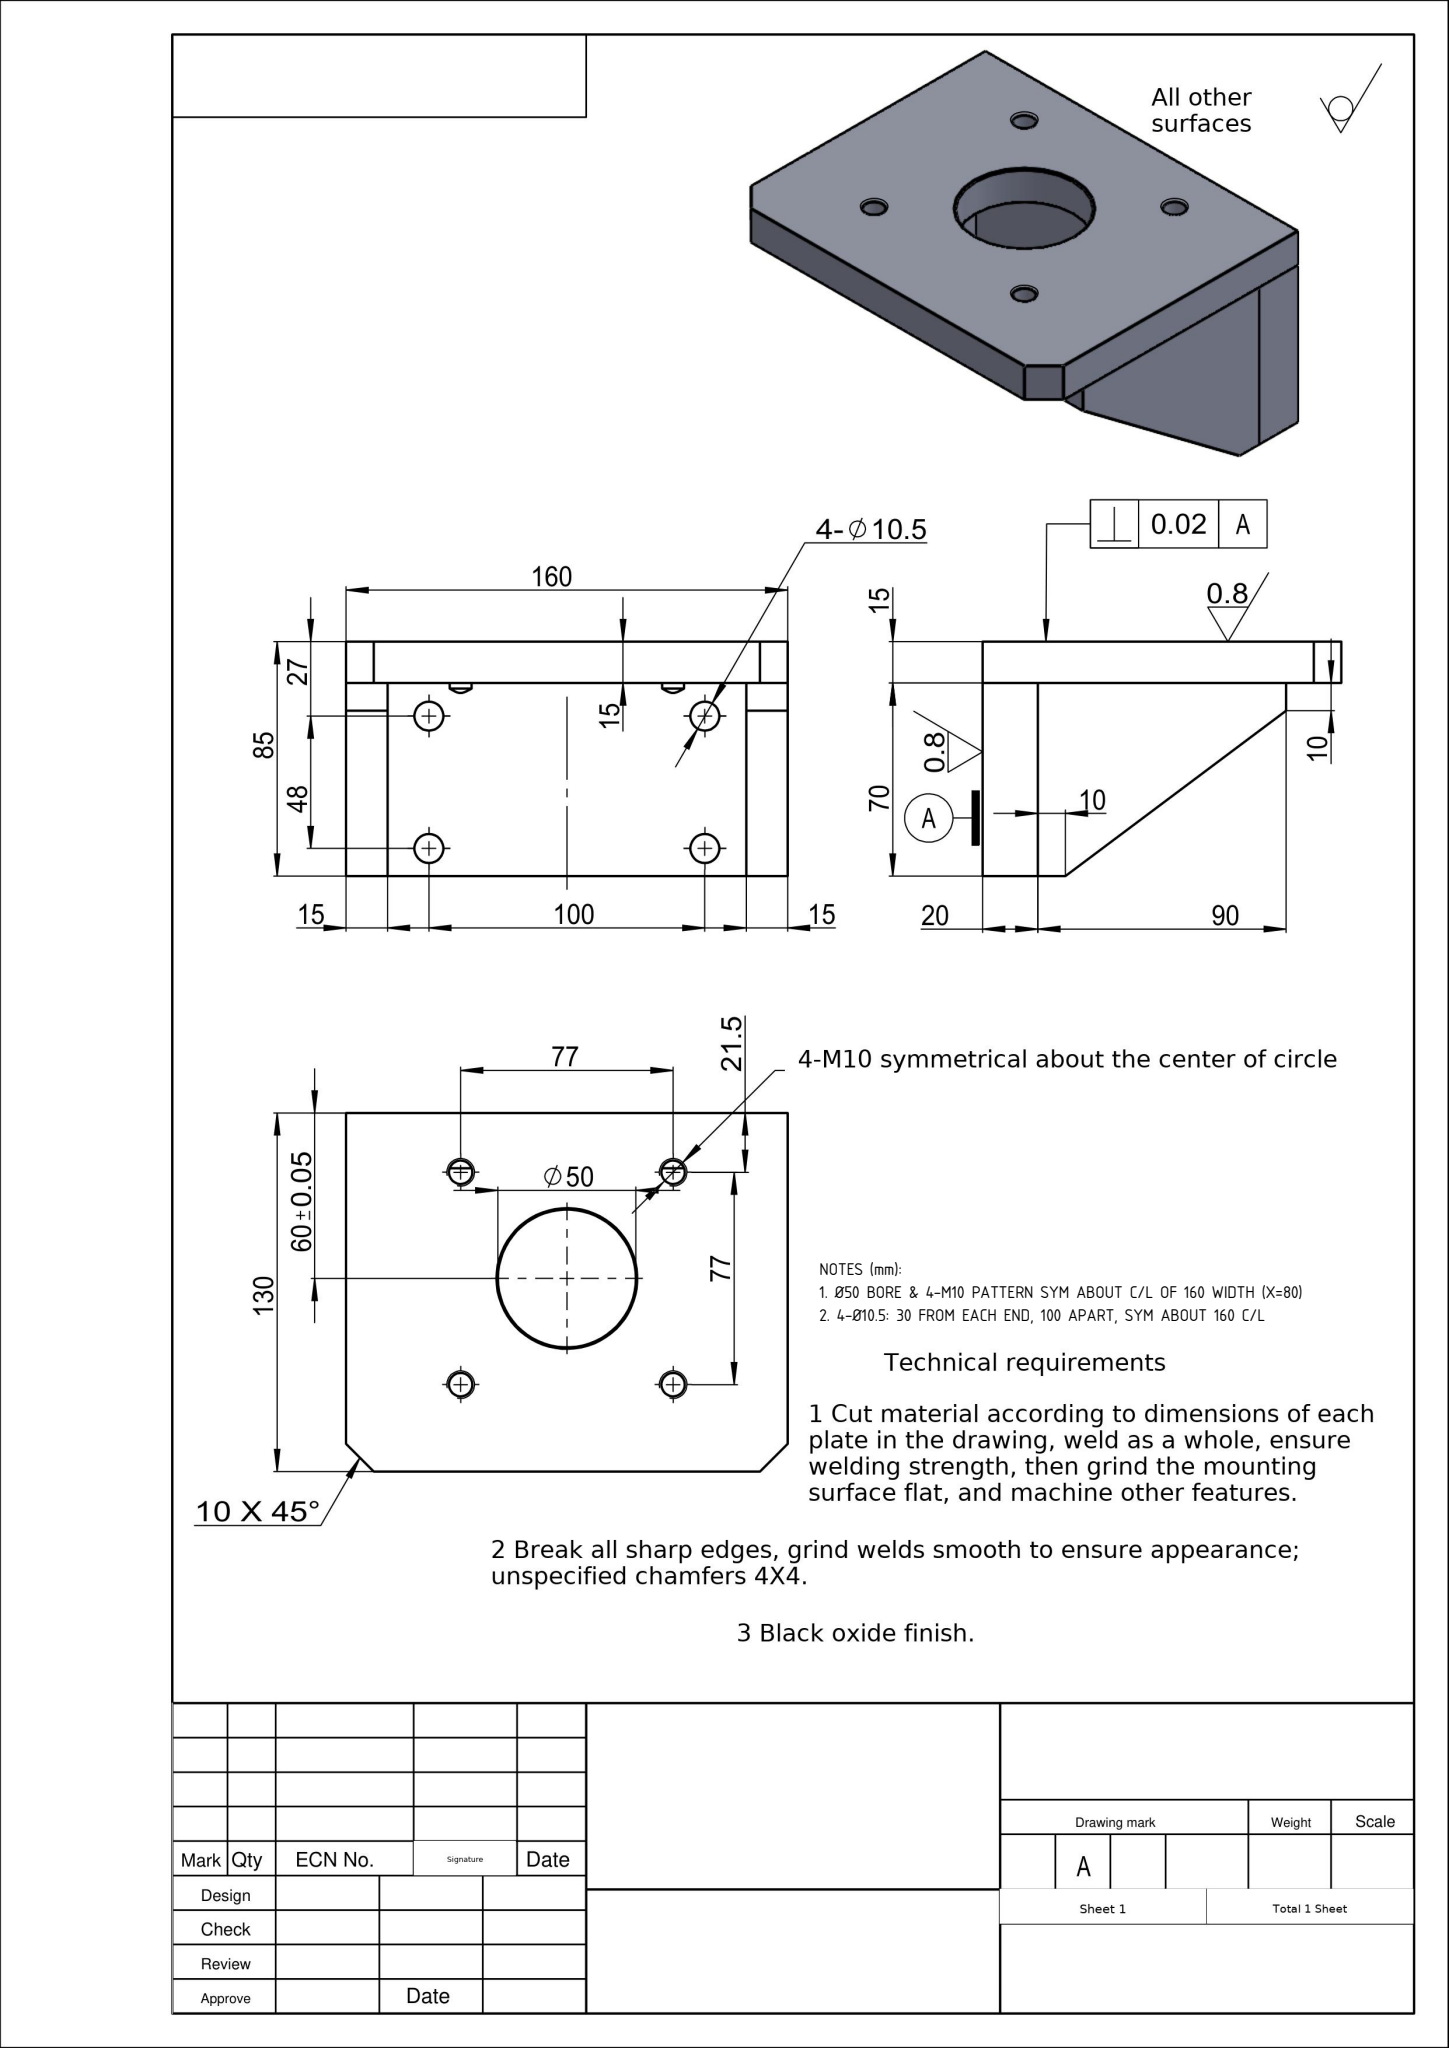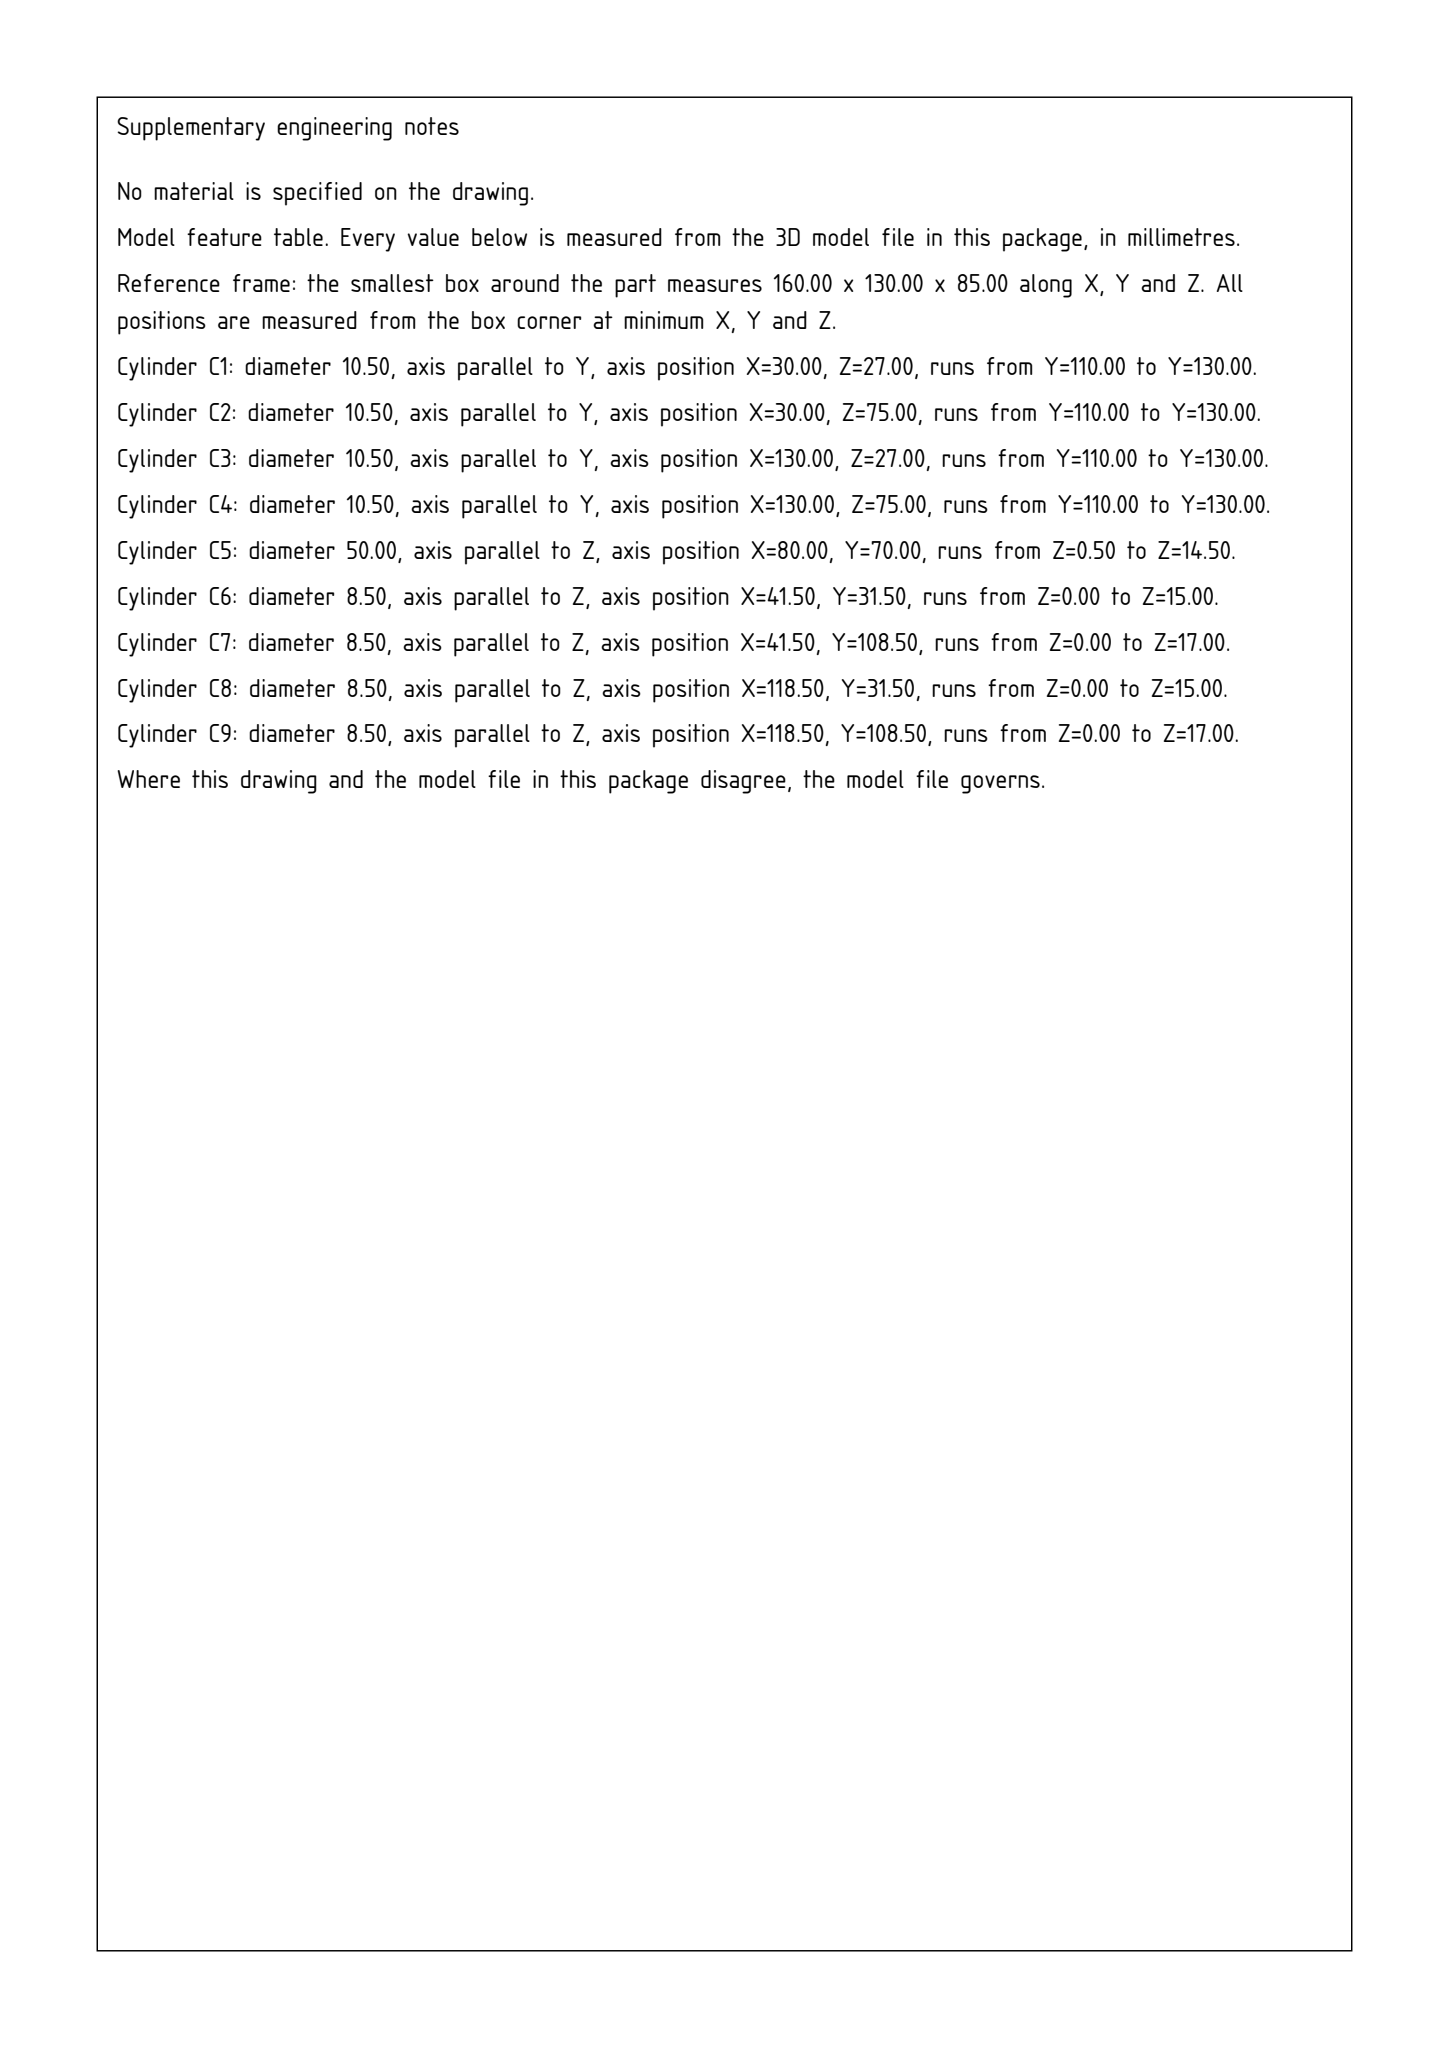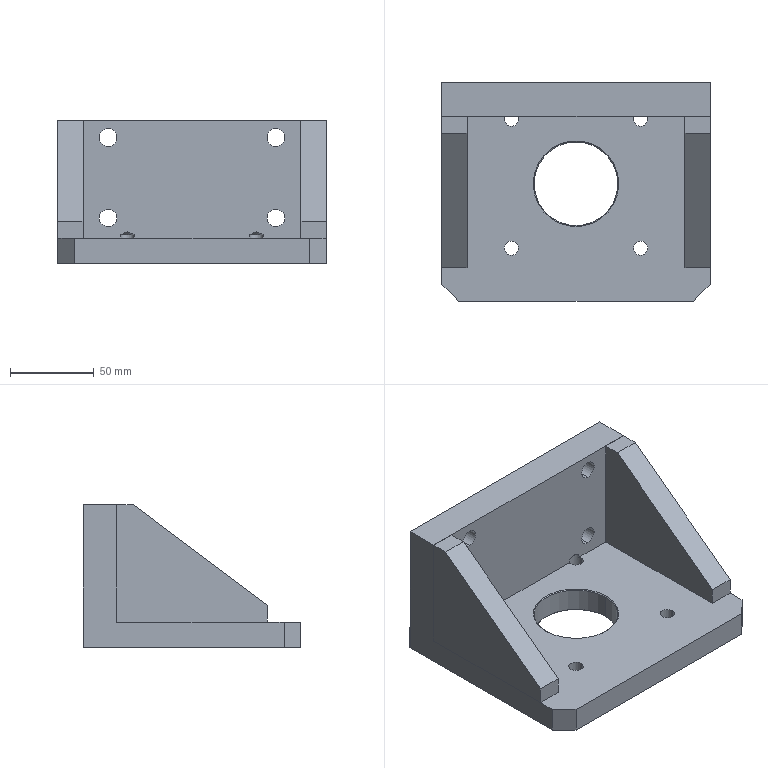Part | SolidWorks | mm | 1 solid | 49 faces | box 160 x 130 x 85 mm | volume 611593 mm3 | plane 25 | cylinder 18 | cone 6 | commonest cylinder face diameters 8.5 x8 10.5 x8 50 x2
Drawing notes:
Ø50 BORE & 4-M10 PATTERN SYM ABOUT C/L OF 160 WIDTH (X=80) | from the solid: Ø50 cyl axis at x=80.0 = 160.001/2; M10 holes at x=41.5 & 118.5 (77 apart, mean 80)
4-Ø10.5: 30 FROM EACH END, 100 APART, SYM ABOUT 160 C/L | from the solid: Ø10.5 cyls at x=30.0 and x=130.0 on 160.001 wide bbox